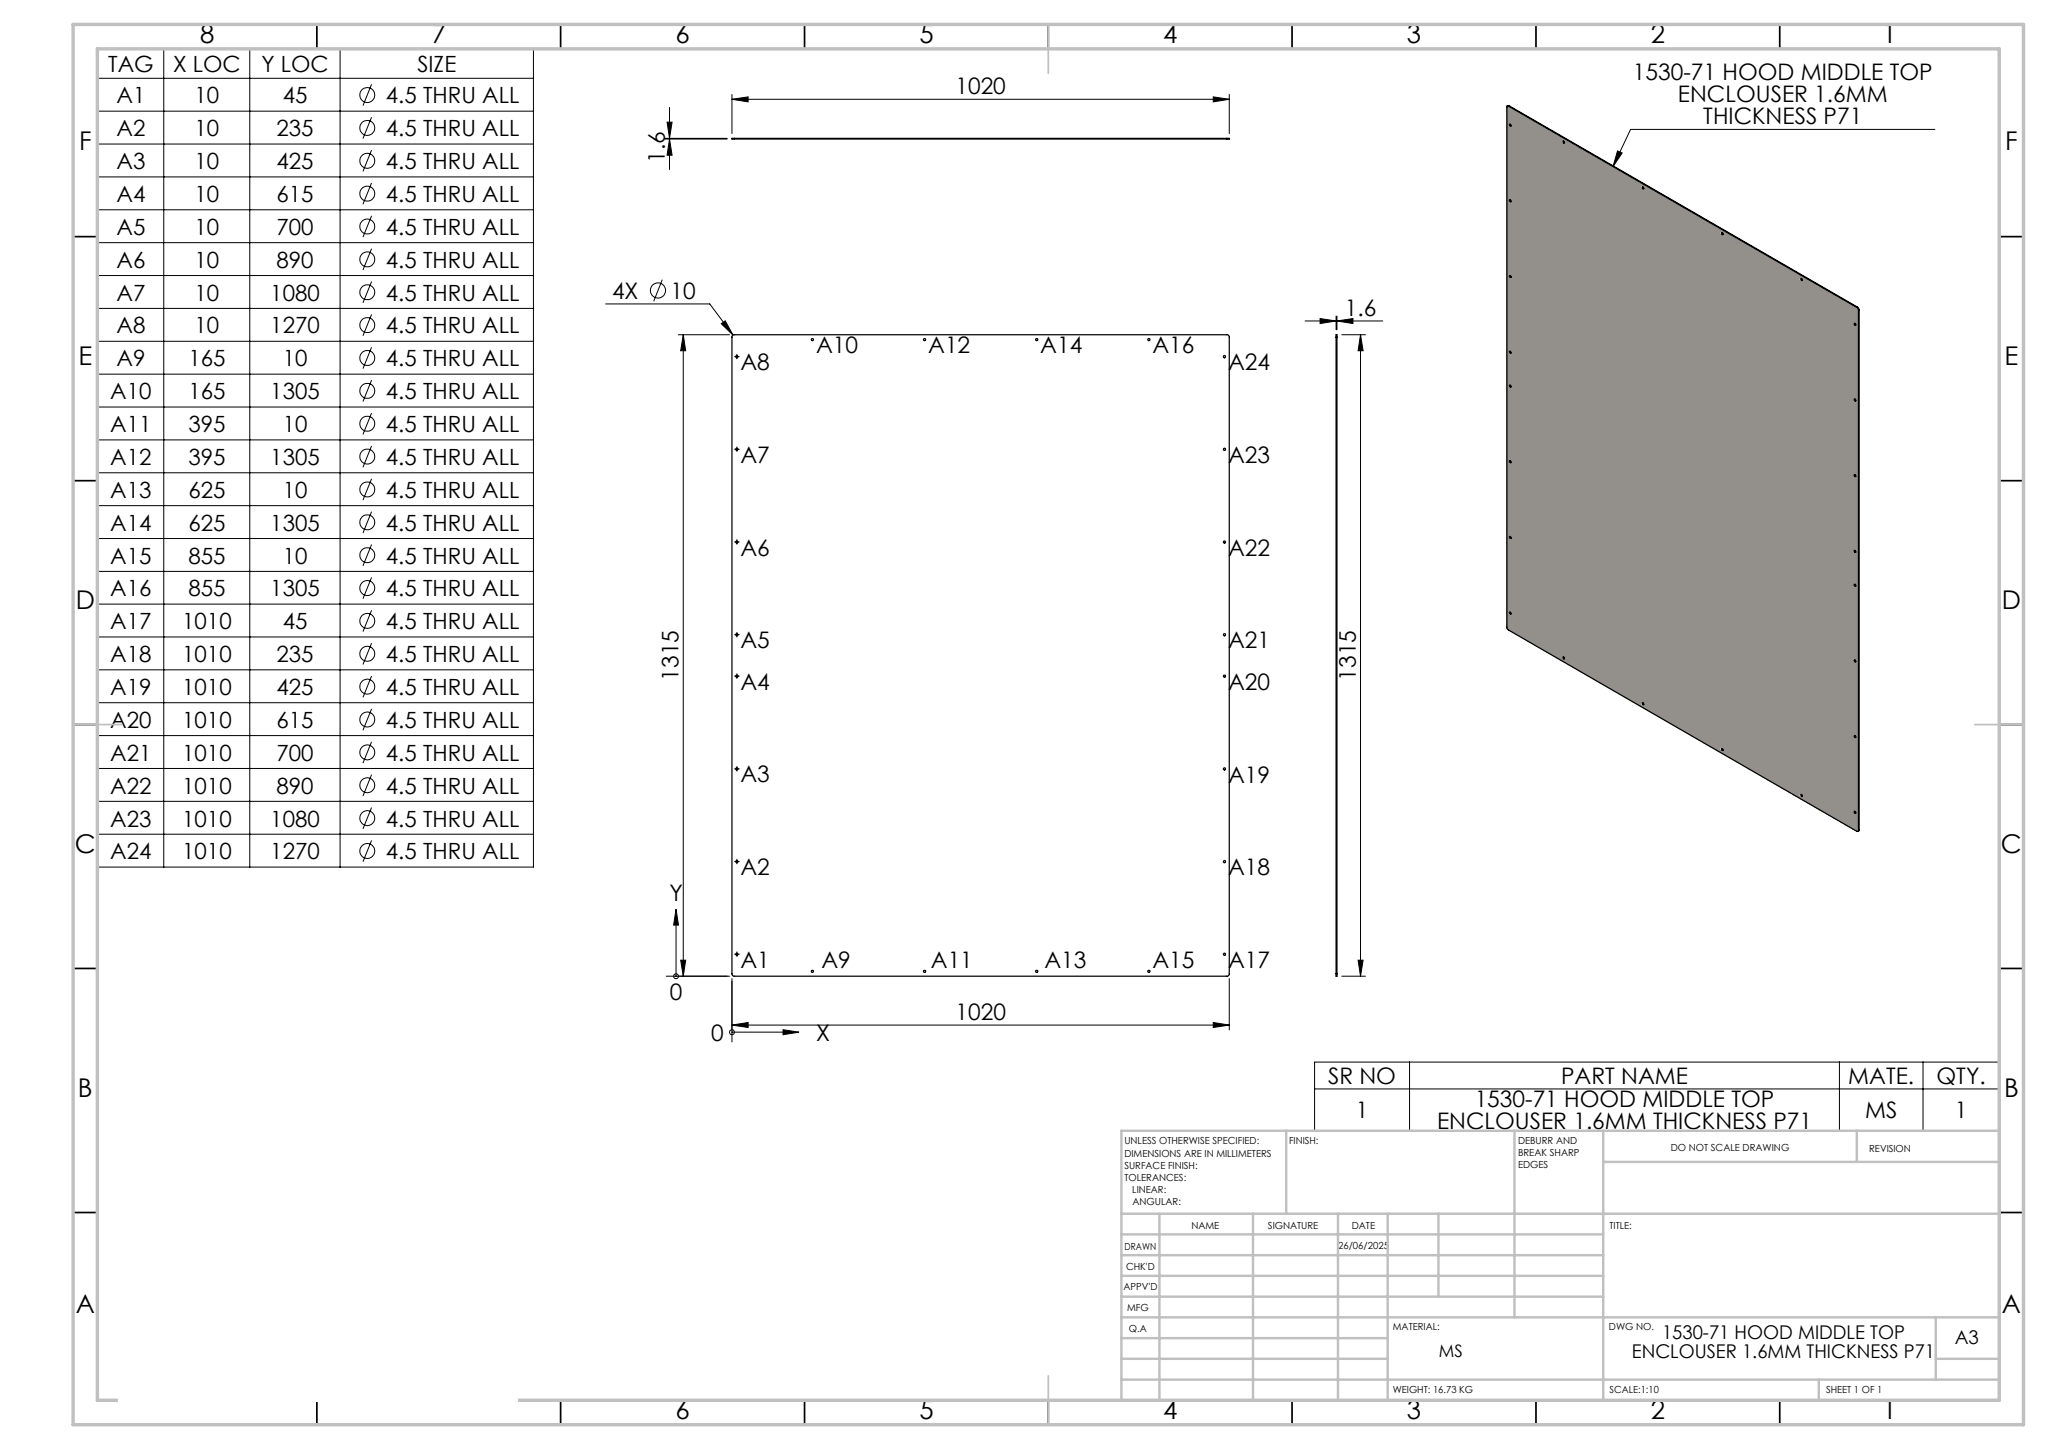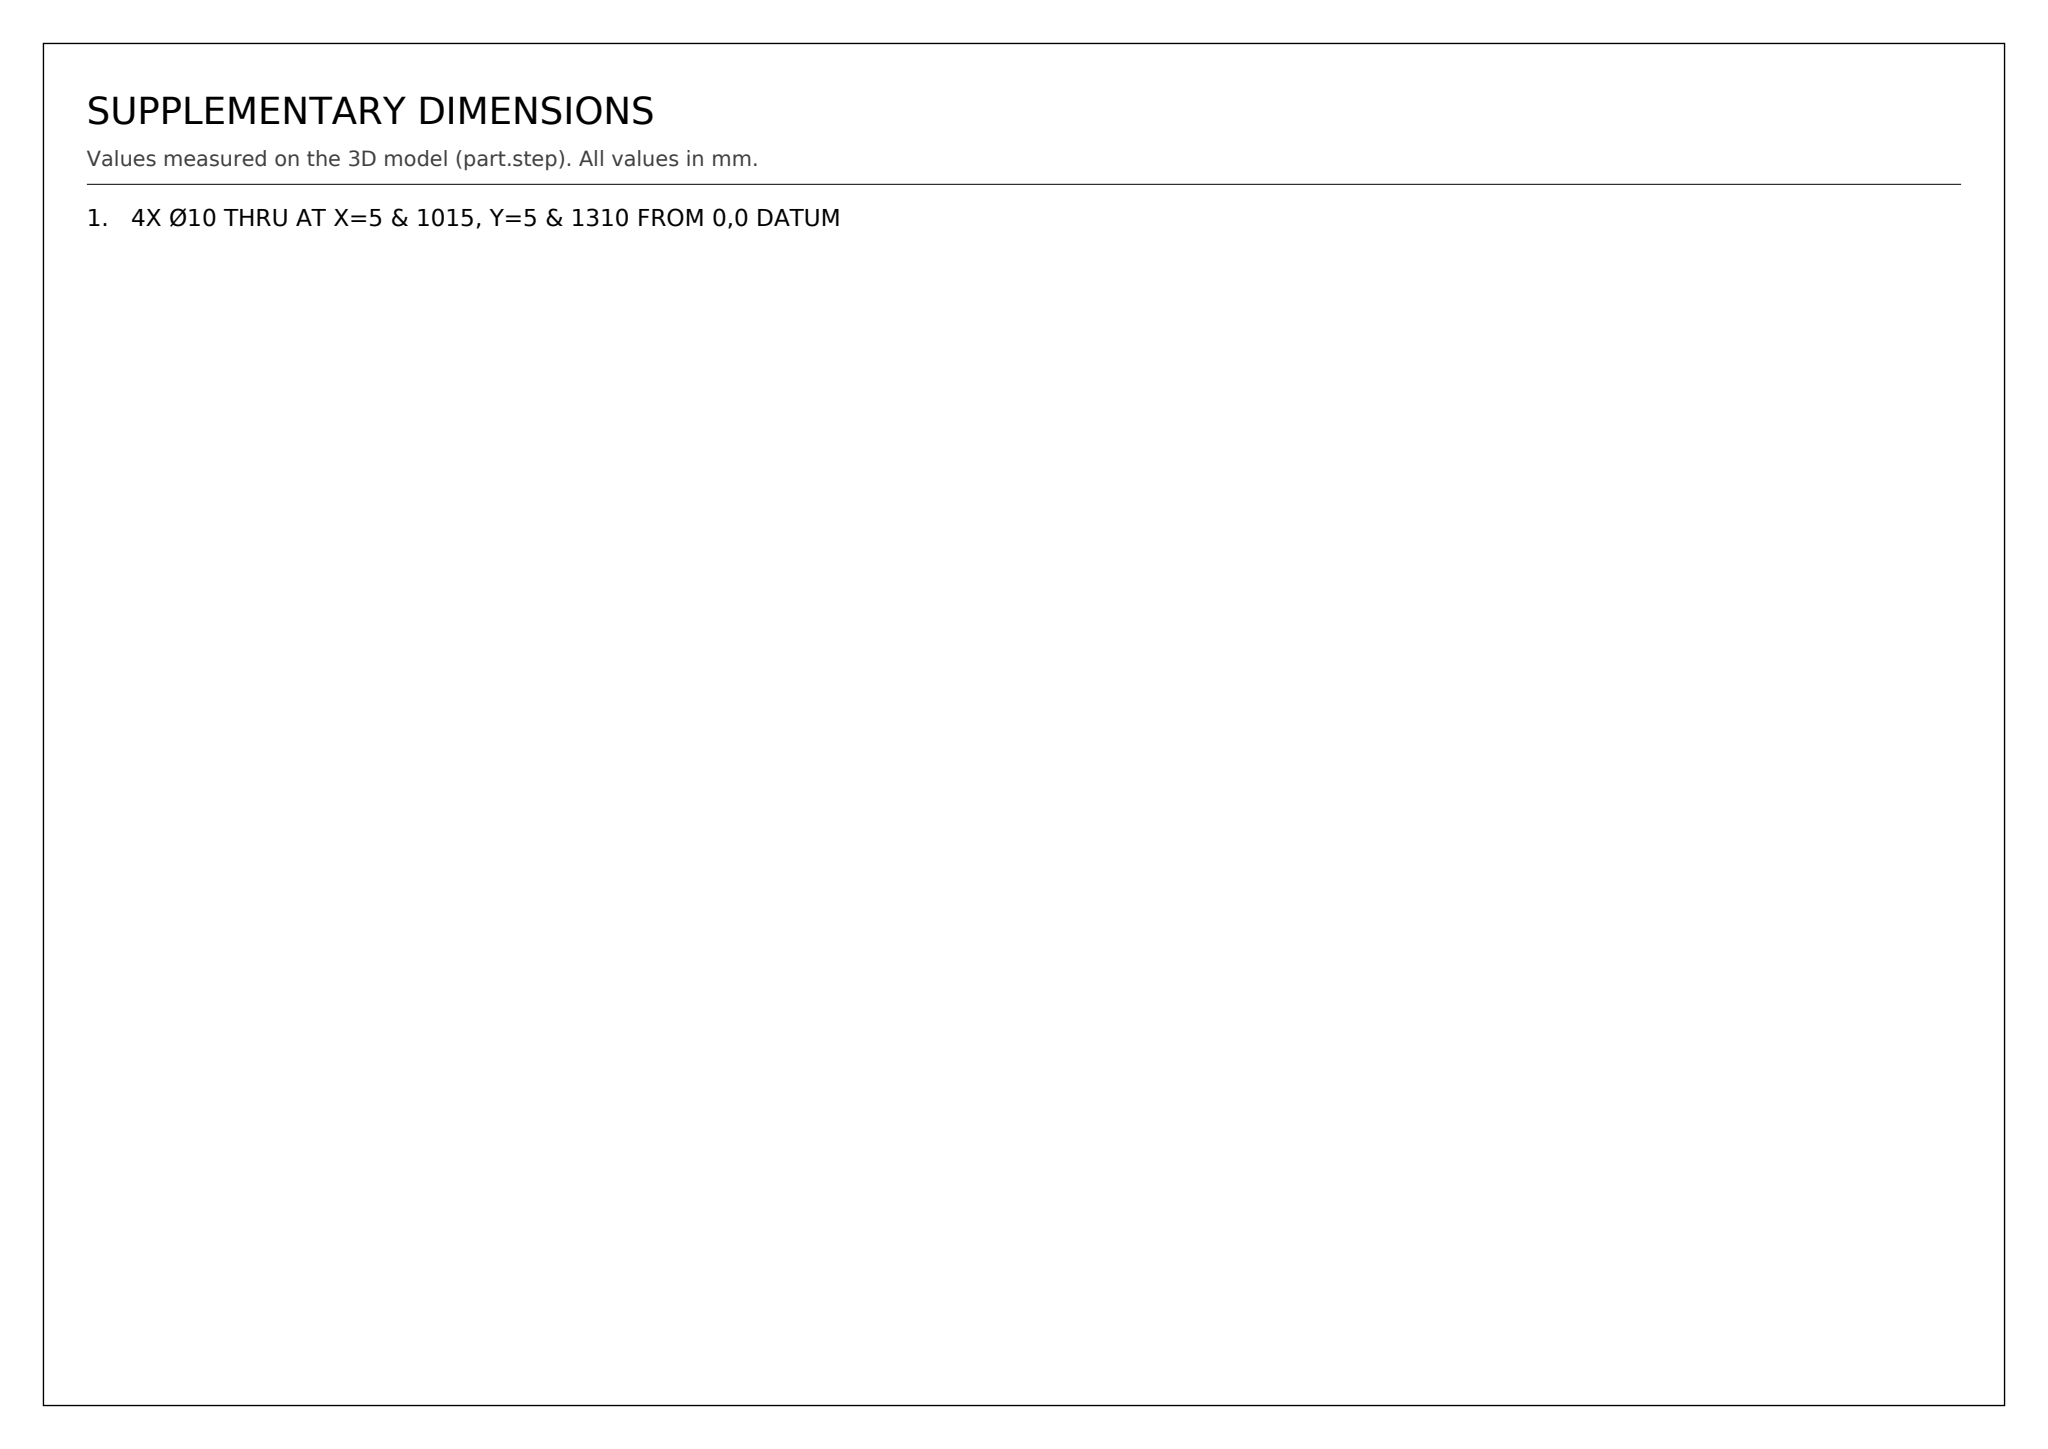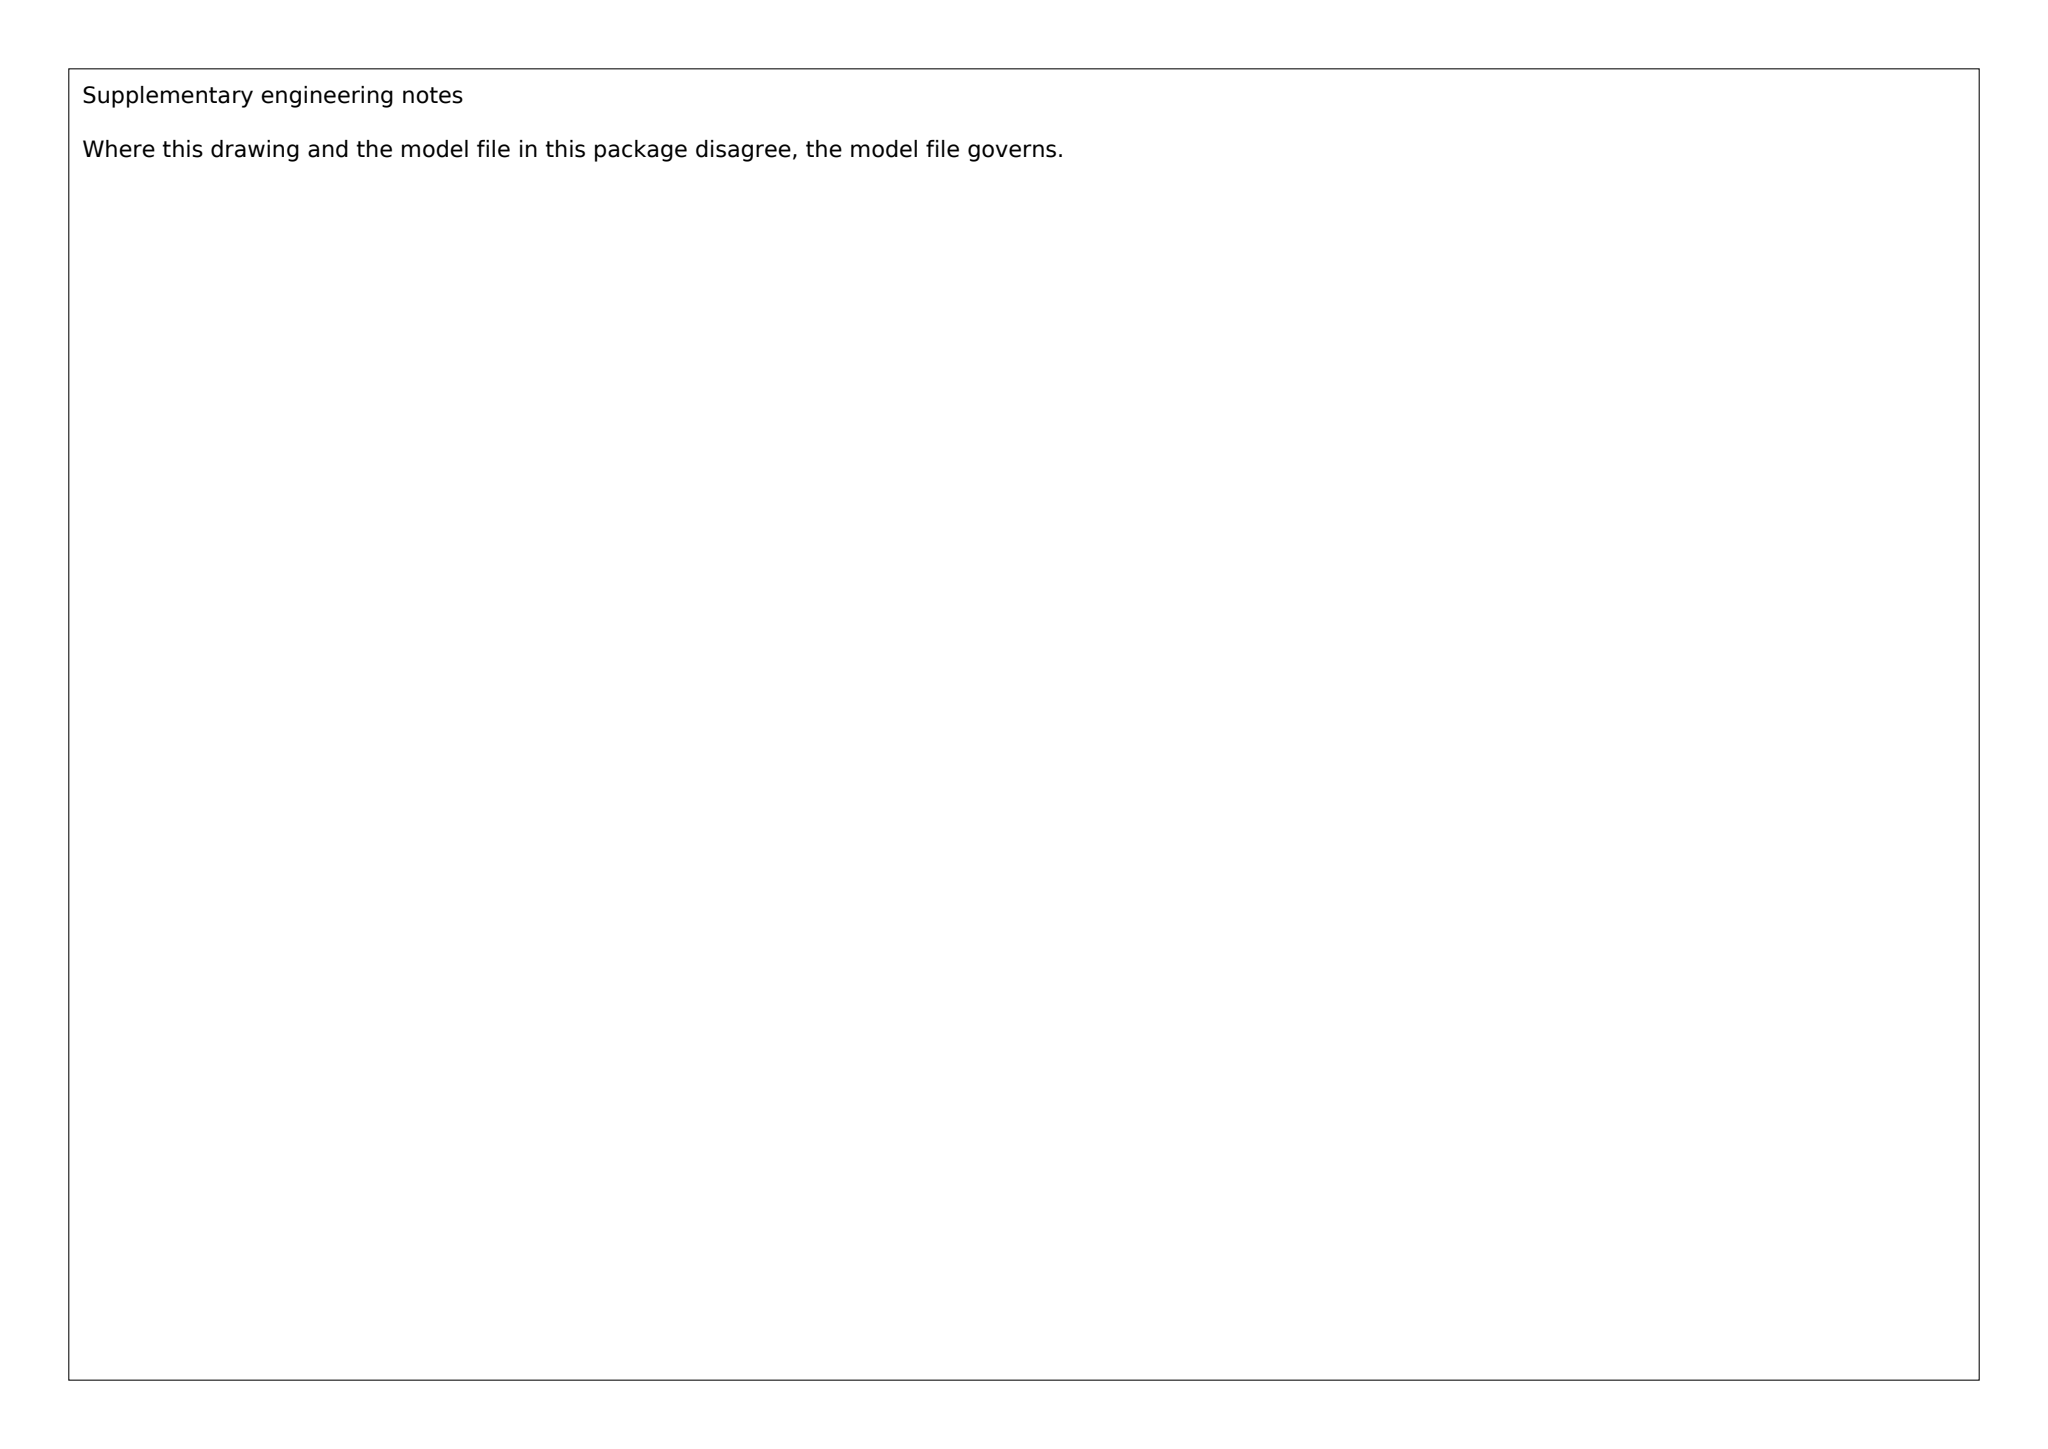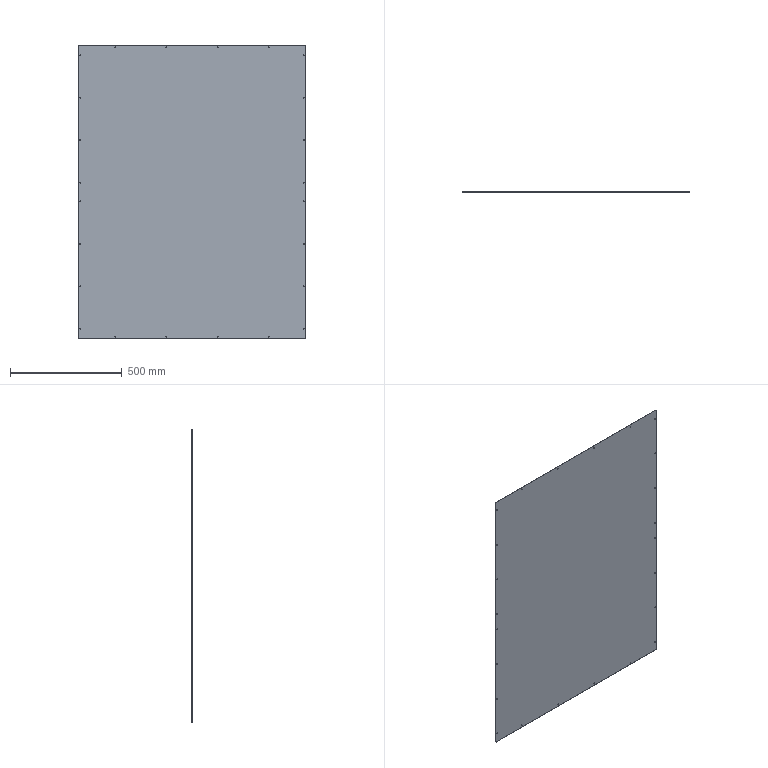Part | SolidWorks | mm | 1 solid | 58 faces | box 1020 x 1.6 x 1315 mm | volume 2145435 mm3 | cylinder 52 | plane 6 | commonest cylinder face diameters 4.5 x48 10 x4
Drawing notes:
4X Ø10 THRU AT X=5 & 1015, Y=5 & 1310 FROM 0,0 DATUM | from the solid: 4 cylinders dia 10, axis y, at (5,5),(5,1310),(1015,5),(1015,1310), len 1.6